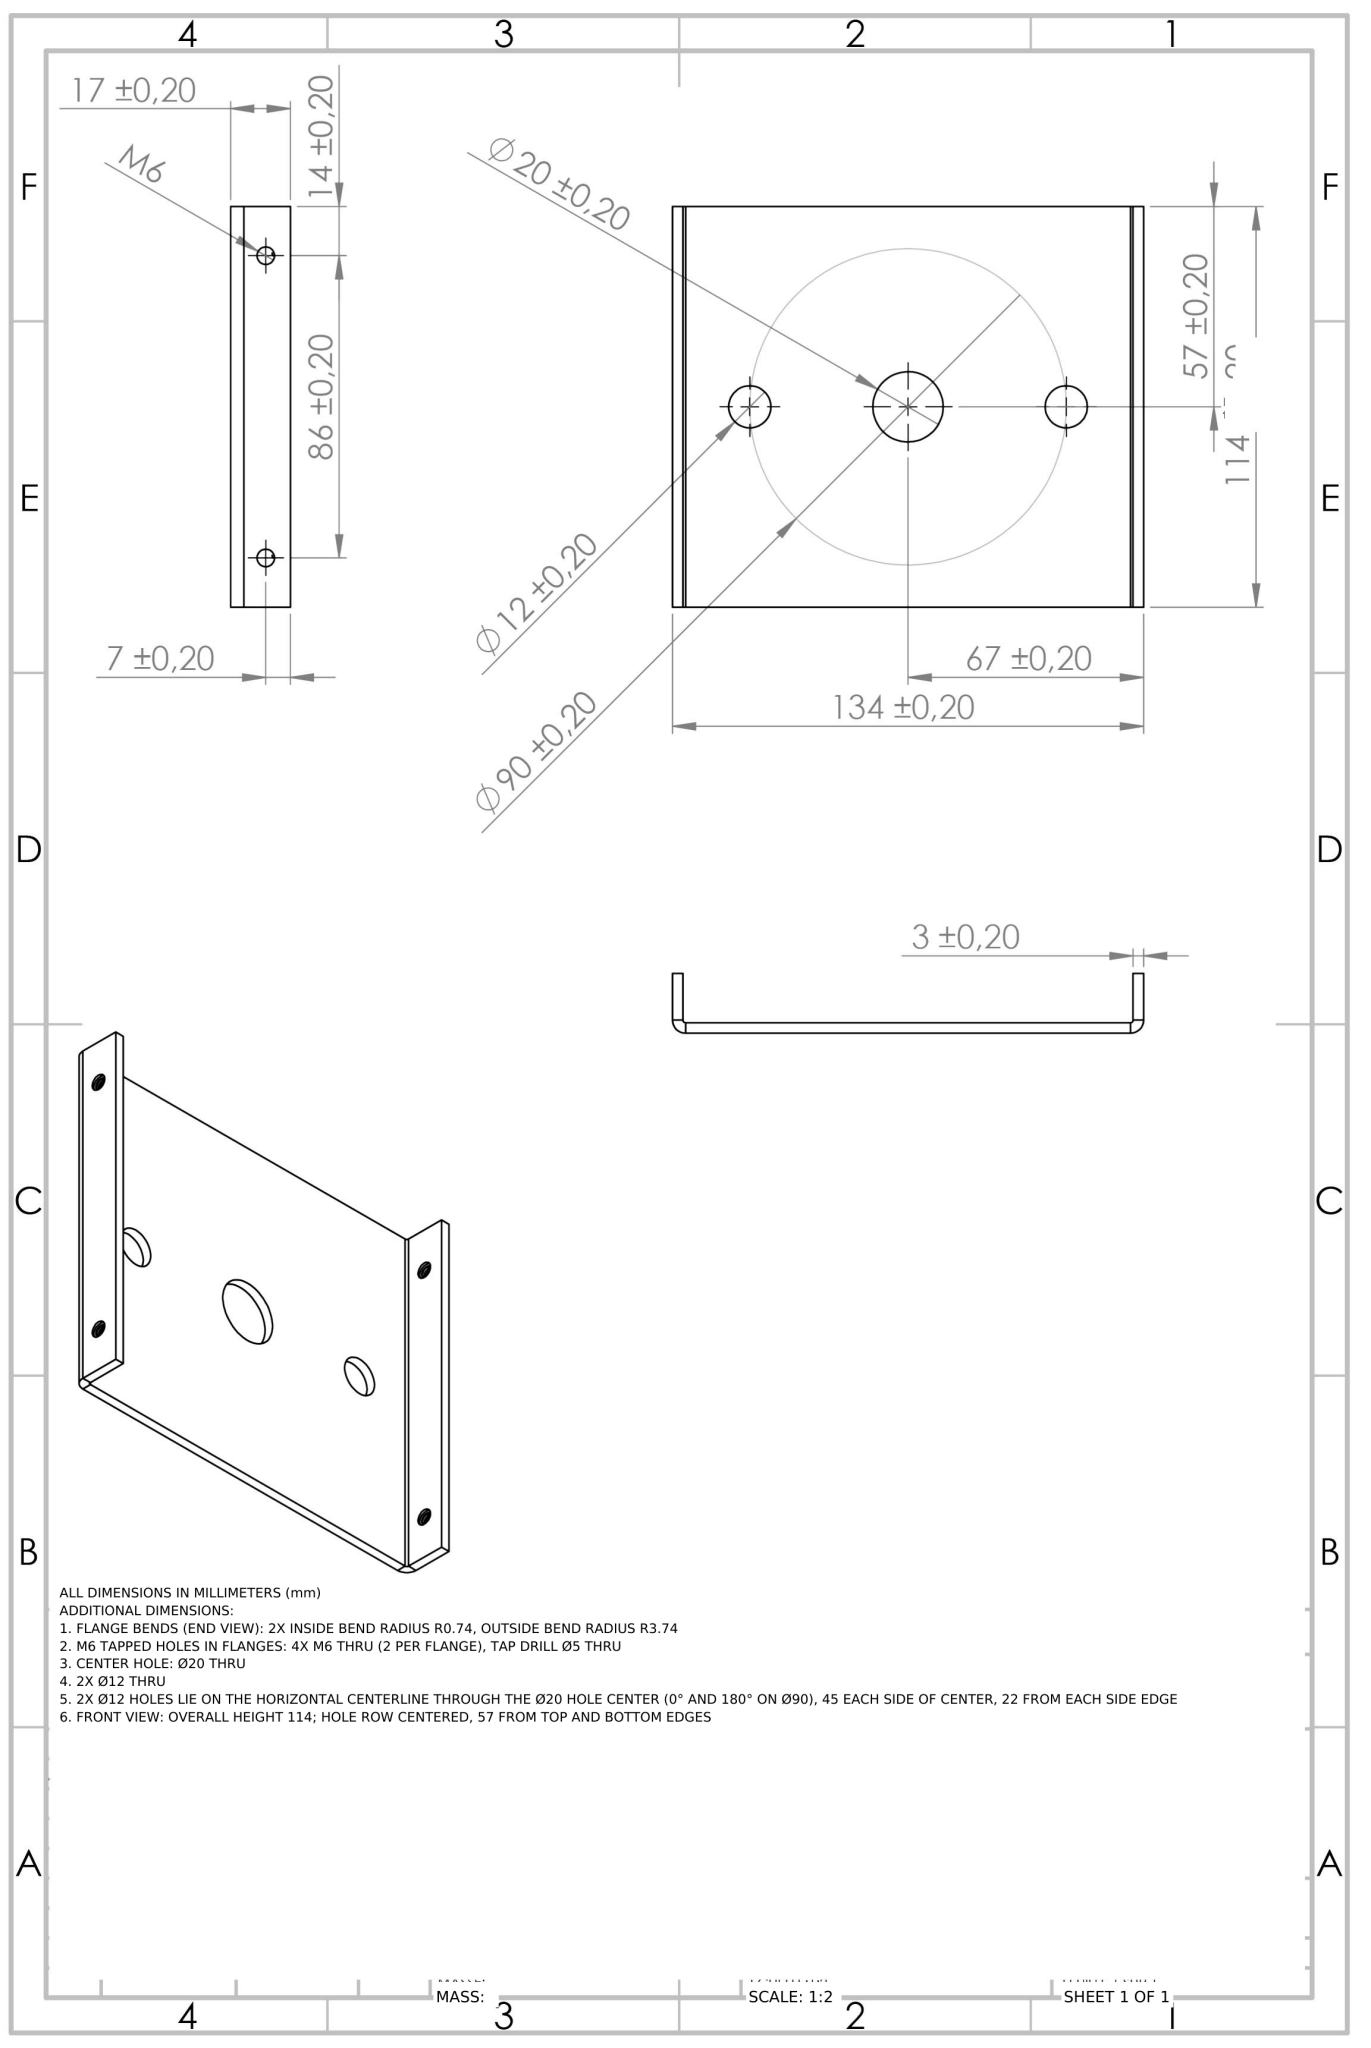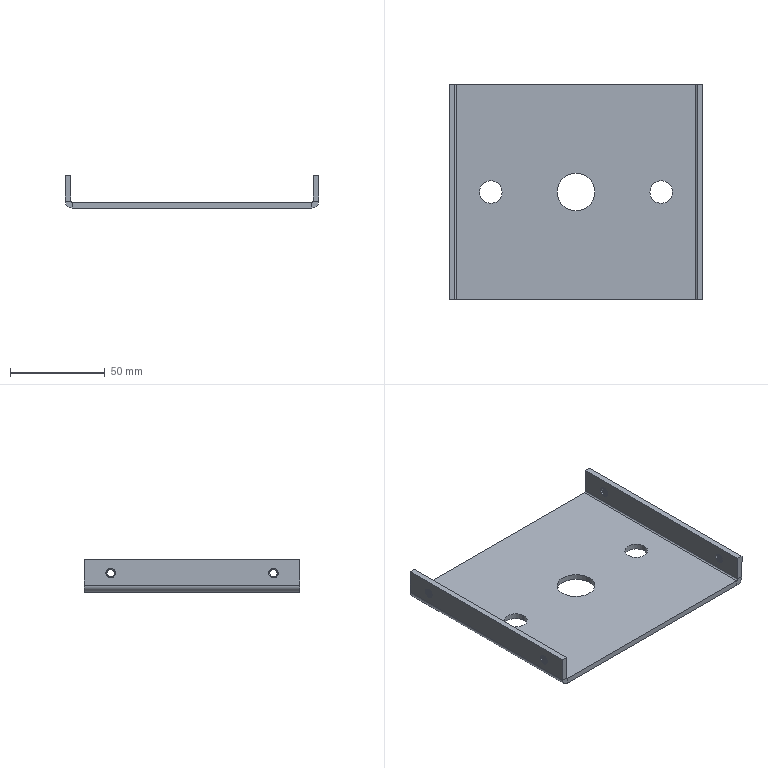Part | NX | mm | 1 solid | 72 faces | box 134 x 114 x 17 mm | volume 52926 mm3 | cylinder 34 | plane 26 | spline 12 | commonest cylinder face diameters 5 x24 12 x4 20 x2 7.473 x2 1.473 x2